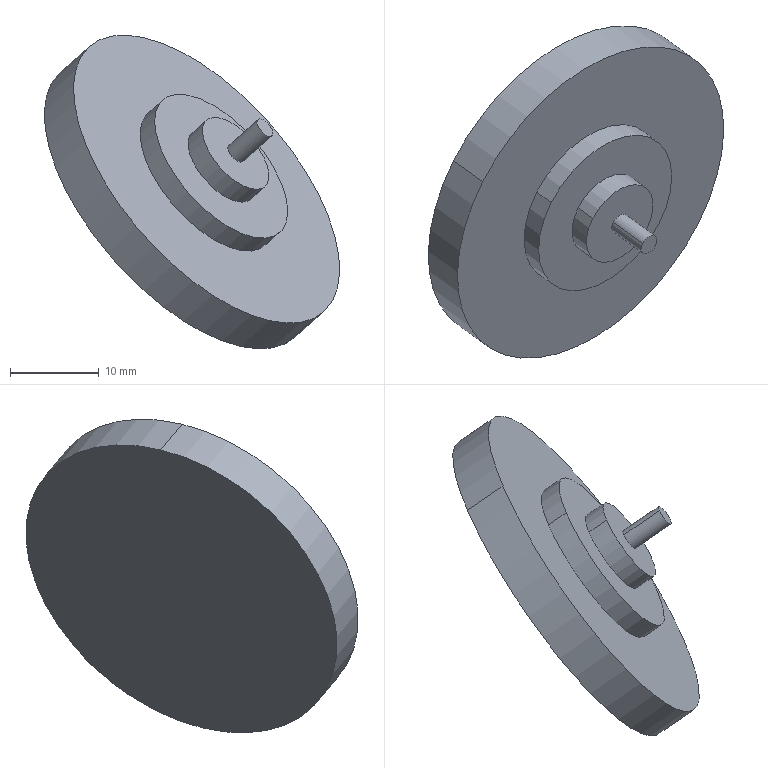Component | SolidWorks | ConnectingPlate-1 | 1 solid | 13 faces | box 33.37 x 37.55 x 35.44 mm | volume 7288 mm3 | cylinder 8 | plane 5 | commonest cylinder face diameters 2.4 x2 10 x2 20 x2 40 x2 | material Copper
build123d program:
from build123d import *

# Parameters (mm, degrees)
SKETCH2_R           = 20
BOSS_EXTRUDE1_DEPTH = 5
SKETCH2_4_R         = 10
BOSS_EXTRUDE2_DEPTH = 2.5
SKETCH2_5_R         = 5
BOSS_EXTRUDE3_DEPTH = 5
SKETCH2_6_R         = 1.2
BOSS_EXTRUDE4_DEPTH = 10


with BuildPart() as part:
    # Sketch2 → Boss-Extrude1 (new body)
    with BuildSketch(Plane(origin=(0, 0, 0), x_dir=(1, 0, 0), z_dir=(0, 1, 0))):
        with Locations(Location((0, 0, 0), (0, 0, 270))):
            Circle(SKETCH2_R)
    extrude(amount=BOSS_EXTRUDE1_DEPTH)

    # Sketch2_4 → Boss-Extrude2 (add)
    with BuildSketch(Plane(origin=(0, 0, 0), x_dir=(1, 0, 0), z_dir=(0, 1, 0))):
        with Locations(Location((0, 0, 0), (0, 0, 270))):
            Circle(SKETCH2_4_R)
    extrude(amount=-BOSS_EXTRUDE2_DEPTH)

    # Sketch2_5 → Boss-Extrude3 (add)
    with BuildSketch(Plane(origin=(0, 0, 0), x_dir=(1, 0, 0), z_dir=(0, 1, 0))):
        with Locations(Location((0, 0, 0), (0, 0, 270))):
            Circle(SKETCH2_5_R)
    extrude(amount=-BOSS_EXTRUDE3_DEPTH)

    # Sketch2_6 → Boss-Extrude4 (add)
    with BuildSketch(Plane(origin=(0, 0, 0), x_dir=(1, 0, 0), z_dir=(0, 1, 0))):
        with Locations(Location((0, 0, 0), (0, 0, 270))):
            Circle(SKETCH2_6_R)
    extrude(amount=-BOSS_EXTRUDE4_DEPTH)


solid = part.part

# Placed as in the assembly
solid = solid.moved(Location((-327.305, -1538.595, -15.587), (-73.169, 23.56, 45.986)))
STEP:
#1=COLOUR_RGB('',0.7922,0.8196,0.9333);
#2=FILL_AREA_STYLE_COLOUR('',#1);
#3=FILL_AREA_STYLE('',(#2));
#4=SURFACE_STYLE_FILL_AREA(#3);
#5=SURFACE_SIDE_STYLE('',(#4));
#6=SURFACE_STYLE_USAGE(.BOTH.,#5);
#7=PRESENTATION_STYLE_ASSIGNMENT((#6));
#8=CARTESIAN_POINT('',(-12.598,-60.768,-0.4217));
#9=VERTEX_POINT('',#8);
#10=CARTESIAN_POINT('',(-12.655,-60.757,-0.3475));
#11=VERTEX_POINT('',#10);
#12=CARTESIAN_POINT('',(-12.626,-60.762,-0.3846));
#13=DIRECTION('',(-0.6592,0.4763,-0.5818));
#14=DIRECTION('',(0.6087,-0.1163,-0.7848));
#15=AXIS2_PLACEMENT_3D('',#12,#13,#14);
#16=CIRCLE('',#15,0.04724);
#17=EDGE_CURVE('',#9,#11,#16,.T.);
#18=ORIENTED_EDGE('',*,*,#17,.T.);
#19=CARTESIAN_POINT('',(-12.785,-60.663,-0.4621));
#20=VERTEX_POINT('',#19);
#21=CARTESIAN_POINT('',(-12.655,-60.757,-0.3475));
#22=DIRECTION('',(-0.6592,0.4763,-0.5818));
#23=VECTOR('',#22,39.37);
#24=LINE('',#21,#23);
#25=EDGE_CURVE('',#11,#20,#24,.T.);
#26=ORIENTED_EDGE('',*,*,#25,.T.);
#27=CARTESIAN_POINT('',(-12.727,-60.674,-0.5362));
#28=VERTEX_POINT('',#27);
#29=CARTESIAN_POINT('',(-12.756,-60.668,-0.4991));
#30=DIRECTION('',(-0.6592,0.4763,-0.5818));
#31=DIRECTION('',(0.6087,-0.1163,-0.7848));
#32=AXIS2_PLACEMENT_3D('',#29,#30,#31);
#33=CIRCLE('',#32,0.04724);
#34=EDGE_CURVE('',#28,#20,#33,.T.);
#35=ORIENTED_EDGE('',*,*,#34,.F.);
#36=CARTESIAN_POINT('',(-12.598,-60.768,-0.4217));
#37=DIRECTION('',(-0.6592,0.4763,-0.5818));
#38=VECTOR('',#37,39.37);
#39=LINE('',#36,#38);
#40=EDGE_CURVE('',#9,#28,#39,.T.);
#41=ORIENTED_EDGE('',*,*,#40,.F.);
#42=EDGE_LOOP('',(#18,#26,#35,#41));
#43=FACE_OUTER_BOUND('',#42,.T.);
#44=CARTESIAN_POINT('',(-12.626,-60.762,-0.3846));
#45=DIRECTION('',(-0.6592,0.4763,-0.5818));
#46=DIRECTION('',(0.6087,-0.1163,-0.7848));
#47=AXIS2_PLACEMENT_3D('',#44,#45,#46);
#48=CYLINDRICAL_SURFACE('',#47,0.04724);
#49=ADVANCED_FACE('',(#43),#48,.T.);
#50=CARTESIAN_POINT('',(-12.636,-60.691,-0.6536));
#51=VERTEX_POINT('',#50);
#52=CARTESIAN_POINT('',(-12.876,-60.645,-0.3446));
#53=VERTEX_POINT('',#52);
#54=CARTESIAN_POINT('',(-12.756,-60.668,-0.4991));
#55=DIRECTION('',(-0.6592,0.4763,-0.5818));
#56=DIRECTION('',(0.6087,-0.1163,-0.7848));
#57=AXIS2_PLACEMENT_3D('',#54,#55,#56);
#58=CIRCLE('',#57,0.1969);
#59=EDGE_CURVE('',#51,#53,#58,.T.);
#60=ORIENTED_EDGE('',*,*,#59,.T.);
#61=CARTESIAN_POINT('',(-12.941,-60.599,-0.4019));
#62=VERTEX_POINT('',#61);
#63=CARTESIAN_POINT('',(-12.876,-60.645,-0.3446));
#64=DIRECTION('',(-0.6592,0.4763,-0.5818));
#65=VECTOR('',#64,39.37);
#66=LINE('',#63,#65);
#67=EDGE_CURVE('',#53,#62,#66,.T.);
#68=ORIENTED_EDGE('',*,*,#67,.T.);
#69=CARTESIAN_POINT('',(-12.701,-60.644,-0.7109));
#70=VERTEX_POINT('',#69);
#71=CARTESIAN_POINT('',(-12.821,-60.622,-0.5564));
#72=DIRECTION('',(-0.6592,0.4763,-0.5818));
#73=DIRECTION('',(0.6087,-0.1163,-0.7848));
#74=AXIS2_PLACEMENT_3D('',#71,#72,#73);
#75=CIRCLE('',#74,0.1969);
#76=EDGE_CURVE('',#70,#62,#75,.T.);
#77=ORIENTED_EDGE('',*,*,#76,.F.);
#78=CARTESIAN_POINT('',(-12.636,-60.691,-0.6536));
#79=DIRECTION('',(-0.6592,0.4763,-0.5818));
#80=VECTOR('',#79,39.37);
#81=LINE('',#78,#80);
#82=EDGE_CURVE('',#51,#70,#81,.T.);
#83=ORIENTED_EDGE('',*,*,#82,.F.);
#84=EDGE_LOOP('',(#60,#68,#77,#83));
#85=FACE_OUTER_BOUND('',#84,.T.);
#86=CARTESIAN_POINT('',(-12.756,-60.668,-0.4991));
#87=DIRECTION('',(-0.6592,0.4763,-0.5818));
#88=DIRECTION('',(0.6087,-0.1163,-0.7848));
#89=AXIS2_PLACEMENT_3D('',#86,#87,#88);
#90=CYLINDRICAL_SURFACE('',#89,0.1969);
#91=ADVANCED_FACE('',(#85),#90,.T.);
#92=CARTESIAN_POINT('',(-12.581,-60.667,-0.8654));
#93=VERTEX_POINT('',#92);
#94=CARTESIAN_POINT('',(-13.061,-60.576,-0.2474));
#95=VERTEX_POINT('',#94);
#96=CARTESIAN_POINT('',(-12.821,-60.622,-0.5564));
#97=DIRECTION('',(-0.6592,0.4763,-0.5818));
#98=DIRECTION('',(0.6087,-0.1163,-0.7848));
#99=AXIS2_PLACEMENT_3D('',#96,#97,#98);
#100=CIRCLE('',#99,0.3937);
#101=EDGE_CURVE('',#93,#95,#100,.T.);
#102=ORIENTED_EDGE('',*,*,#101,.T.);
#103=CARTESIAN_POINT('',(-13.126,-60.529,-0.3047));
#104=VERTEX_POINT('',#103);
#105=CARTESIAN_POINT('',(-13.061,-60.576,-0.2474));
#106=DIRECTION('',(-0.6592,0.4763,-0.5818));
#107=VECTOR('',#106,39.37);
#108=LINE('',#105,#107);
#109=EDGE_CURVE('',#95,#104,#108,.T.);
#110=ORIENTED_EDGE('',*,*,#109,.T.);
#111=CARTESIAN_POINT('',(-12.646,-60.62,-0.9227));
#112=VERTEX_POINT('',#111);
#113=CARTESIAN_POINT('',(-12.886,-60.575,-0.6137));
#114=DIRECTION('',(-0.6592,0.4763,-0.5818));
#115=DIRECTION('',(0.6087,-0.1163,-0.7848));
#116=AXIS2_PLACEMENT_3D('',#113,#114,#115);
#117=CIRCLE('',#116,0.3937);
#118=EDGE_CURVE('',#112,#104,#117,.T.);
#119=ORIENTED_EDGE('',*,*,#118,.F.);
#120=CARTESIAN_POINT('',(-12.581,-60.667,-0.8654));
#121=DIRECTION('',(-0.6592,0.4763,-0.5818));
#122=VECTOR('',#121,39.37);
#123=LINE('',#120,#122);
#124=EDGE_CURVE('',#93,#112,#123,.T.);
#125=ORIENTED_EDGE('',*,*,#124,.F.);
#126=EDGE_LOOP('',(#102,#110,#119,#125));
#127=FACE_OUTER_BOUND('',#126,.T.);
#128=CARTESIAN_POINT('',(-12.821,-60.622,-0.5564));
#129=DIRECTION('',(-0.6592,0.4763,-0.5818));
#130=DIRECTION('',(0.6087,-0.1163,-0.7848));
#131=AXIS2_PLACEMENT_3D('',#128,#129,#130);
#132=CYLINDRICAL_SURFACE('',#131,0.3937);
#133=ADVANCED_FACE('',(#127),#132,.T.);
#134=CARTESIAN_POINT('',(-12.536,-60.572,-1.346));
#135=VERTEX_POINT('',#134);
#136=CARTESIAN_POINT('',(-13.495,-60.389,-0.1102));
#137=VERTEX_POINT('',#136);
#138=CARTESIAN_POINT('',(-13.016,-60.481,-0.7282));
#139=DIRECTION('',(-0.6592,0.4763,-0.5818));
#140=DIRECTION('',(0.6087,-0.1163,-0.7848));
#141=AXIS2_PLACEMENT_3D('',#138,#139,#140);
#142=CIRCLE('',#141,0.7874);
#143=EDGE_CURVE('',#135,#137,#142,.T.);
#144=ORIENTED_EDGE('',*,*,#143,.F.);
#145=CARTESIAN_POINT('',(-12.407,-60.666,-1.232));
#146=VERTEX_POINT('',#145);
#147=CARTESIAN_POINT('',(-12.536,-60.572,-1.346));
#148=DIRECTION('',(0.6592,-0.4763,0.5818));
#149=VECTOR('',#148,39.37);
#150=LINE('',#147,#149);
#151=EDGE_CURVE('',#135,#146,#150,.T.);
#152=ORIENTED_EDGE('',*,*,#151,.T.);
#153=CARTESIAN_POINT('',(-13.365,-60.483,0.00431));
#154=VERTEX_POINT('',#153);
#155=CARTESIAN_POINT('',(-12.886,-60.575,-0.6137));
#156=DIRECTION('',(-0.6592,0.4763,-0.5818));
#157=DIRECTION('',(0.6087,-0.1163,-0.7848));
#158=AXIS2_PLACEMENT_3D('',#155,#156,#157);
#159=CIRCLE('',#158,0.7874);
#160=EDGE_CURVE('',#146,#154,#159,.T.);
#161=ORIENTED_EDGE('',*,*,#160,.T.);
#162=CARTESIAN_POINT('',(-13.495,-60.389,-0.1102));
#163=DIRECTION('',(0.6592,-0.4763,0.5818));
#164=VECTOR('',#163,39.37);
#165=LINE('',#162,#164);
#166=EDGE_CURVE('',#137,#154,#165,.T.);
#167=ORIENTED_EDGE('',*,*,#166,.F.);
#168=EDGE_LOOP('',(#144,#152,#161,#167));
#169=FACE_OUTER_BOUND('',#168,.T.);
#170=CARTESIAN_POINT('',(-13.016,-60.481,-0.7282));
#171=DIRECTION('',(0.6592,-0.4763,0.5818));
#172=DIRECTION('',(-0.6087,0.1163,0.7848));
#173=AXIS2_PLACEMENT_3D('',#170,#171,#172);
#174=CYLINDRICAL_SURFACE('',#173,0.7874);
#175=ADVANCED_FACE('',(#169),#174,.T.);
#176=ORIENTED_EDGE('',*,*,#151,.F.);
#177=CARTESIAN_POINT('',(-13.016,-60.481,-0.7282));
#178=DIRECTION('',(-0.6592,0.4763,-0.5818));
#179=DIRECTION('',(0.6087,-0.1163,-0.7848));
#180=AXIS2_PLACEMENT_3D('',#177,#178,#179);
#181=CIRCLE('',#180,0.7874);
#182=EDGE_CURVE('',#137,#135,#181,.T.);
#183=ORIENTED_EDGE('',*,*,#182,.F.);
#184=ORIENTED_EDGE('',*,*,#166,.T.);
#185=CARTESIAN_POINT('',(-12.886,-60.575,-0.6137));
#186=DIRECTION('',(-0.6592,0.4763,-0.5818));
#187=DIRECTION('',(0.6087,-0.1163,-0.7848));
#188=AXIS2_PLACEMENT_3D('',#185,#186,#187);
#189=CIRCLE('',#188,0.7874);
#190=EDGE_CURVE('',#154,#146,#189,.T.);
#191=ORIENTED_EDGE('',*,*,#190,.T.);
#192=EDGE_LOOP('',(#176,#183,#184,#191));
#193=FACE_OUTER_BOUND('',#192,.T.);
#194=CARTESIAN_POINT('',(-13.016,-60.481,-0.7282));
#195=DIRECTION('',(0.6592,-0.4763,0.5818));
#196=DIRECTION('',(-0.6087,0.1163,0.7848));
#197=AXIS2_PLACEMENT_3D('',#194,#195,#196);
#198=CYLINDRICAL_SURFACE('',#197,0.7874);
#199=ADVANCED_FACE('',(#193),#198,.T.);
#200=ORIENTED_EDGE('',*,*,#182,.T.);
#201=ORIENTED_EDGE('',*,*,#143,.T.);
#202=EDGE_LOOP('',(#200,#201));
#203=FACE_OUTER_BOUND('',#202,.T.);
#204=CARTESIAN_POINT('',(-13.016,-60.481,-0.7282));
#205=DIRECTION('',(-0.6592,0.4763,-0.5818));
#206=DIRECTION('',(0.6087,-0.1163,-0.7848));
#207=AXIS2_PLACEMENT_3D('',#204,#205,#206);
#208=PLANE('',#207);
#209=ADVANCED_FACE('',(#203),#208,.T.);
#210=ORIENTED_EDGE('',*,*,#118,.T.);
#211=CARTESIAN_POINT('',(-12.886,-60.575,-0.6137));
#212=DIRECTION('',(-0.6592,0.4763,-0.5818));
#213=DIRECTION('',(0.6087,-0.1163,-0.7848));
#214=AXIS2_PLACEMENT_3D('',#211,#212,#213);
#215=CIRCLE('',#214,0.3937);
#216=EDGE_CURVE('',#104,#112,#215,.T.);
#217=ORIENTED_EDGE('',*,*,#216,.T.);
#218=EDGE_LOOP('',(#210,#217));
#219=FACE_BOUND('',#218,.T.);
#220=ORIENTED_EDGE('',*,*,#190,.F.);
#221=ORIENTED_EDGE('',*,*,#160,.F.);
#222=EDGE_LOOP('',(#220,#221));
#223=FACE_OUTER_BOUND('',#222,.T.);
#224=CARTESIAN_POINT('',(-12.886,-60.575,-0.6137));
#225=DIRECTION('',(-0.6592,0.4763,-0.5818));
#226=DIRECTION('',(0.6087,-0.1163,-0.7848));
#227=AXIS2_PLACEMENT_3D('',#224,#225,#226);
#228=PLANE('',#227);
#229=ADVANCED_FACE('',(#219,#223),#228,.F.);
#230=ORIENTED_EDGE('',*,*,#109,.F.);
#231=CARTESIAN_POINT('',(-12.821,-60.622,-0.5564));
#232=DIRECTION('',(-0.6592,0.4763,-0.5818));
#233=DIRECTION('',(0.6087,-0.1163,-0.7848));
#234=AXIS2_PLACEMENT_3D('',#231,#232,#233);
#235=CIRCLE('',#234,0.3937);
#236=EDGE_CURVE('',#95,#93,#235,.T.);
#237=ORIENTED_EDGE('',*,*,#236,.T.);
#238=ORIENTED_EDGE('',*,*,#124,.T.);
#239=ORIENTED_EDGE('',*,*,#216,.F.);
#240=EDGE_LOOP('',(#230,#237,#238,#239));
#241=FACE_OUTER_BOUND('',#240,.T.);
#242=CARTESIAN_POINT('',(-12.821,-60.622,-0.5564));
#243=DIRECTION('',(-0.6592,0.4763,-0.5818));
#244=DIRECTION('',(0.6087,-0.1163,-0.7848));
#245=AXIS2_PLACEMENT_3D('',#242,#243,#244);
#246=CYLINDRICAL_SURFACE('',#245,0.3937);
#247=ADVANCED_FACE('',(#241),#246,.T.);
#248=ORIENTED_EDGE('',*,*,#76,.T.);
#249=CARTESIAN_POINT('',(-12.821,-60.622,-0.5564));
#250=DIRECTION('',(-0.6592,0.4763,-0.5818));
#251=DIRECTION('',(0.6087,-0.1163,-0.7848));
#252=AXIS2_PLACEMENT_3D('',#249,#250,#251);
#253=CIRCLE('',#252,0.1969);
#254=EDGE_CURVE('',#62,#70,#253,.T.);
#255=ORIENTED_EDGE('',*,*,#254,.T.);
#256=EDGE_LOOP('',(#248,#255));
#257=FACE_BOUND('',#256,.T.);
#258=ORIENTED_EDGE('',*,*,#101,.F.);
#259=ORIENTED_EDGE('',*,*,#236,.F.);
#260=EDGE_LOOP('',(#258,#259));
#261=FACE_OUTER_BOUND('',#260,.T.);
#262=CARTESIAN_POINT('',(-12.821,-60.622,-0.5564));
#263=DIRECTION('',(-0.6592,0.4763,-0.5818));
#264=DIRECTION('',(0.6087,-0.1163,-0.7848));
#265=AXIS2_PLACEMENT_3D('',#262,#263,#264);
#266=PLANE('',#265);
#267=ADVANCED_FACE('',(#257,#261),#266,.F.);
#268=ORIENTED_EDGE('',*,*,#67,.F.);
#269=CARTESIAN_POINT('',(-12.756,-60.668,-0.4991));
#270=DIRECTION('',(-0.6592,0.4763,-0.5818));
#271=DIRECTION('',(0.6087,-0.1163,-0.7848));
#272=AXIS2_PLACEMENT_3D('',#269,#270,#271);
#273=CIRCLE('',#272,0.1969);
#274=EDGE_CURVE('',#53,#51,#273,.T.);
#275=ORIENTED_EDGE('',*,*,#274,.T.);
#276=ORIENTED_EDGE('',*,*,#82,.T.);
#277=ORIENTED_EDGE('',*,*,#254,.F.);
#278=EDGE_LOOP('',(#268,#275,#276,#277));
#279=FACE_OUTER_BOUND('',#278,.T.);
#280=CARTESIAN_POINT('',(-12.756,-60.668,-0.4991));
#281=DIRECTION('',(-0.6592,0.4763,-0.5818));
#282=DIRECTION('',(0.6087,-0.1163,-0.7848));
#283=AXIS2_PLACEMENT_3D('',#280,#281,#282);
#284=CYLINDRICAL_SURFACE('',#283,0.1969);
#285=ADVANCED_FACE('',(#279),#284,.T.);
#286=ORIENTED_EDGE('',*,*,#34,.T.);
#287=CARTESIAN_POINT('',(-12.756,-60.668,-0.4991));
#288=DIRECTION('',(-0.6592,0.4763,-0.5818));
#289=DIRECTION('',(0.6087,-0.1163,-0.7848));
#290=AXIS2_PLACEMENT_3D('',#287,#288,#289);
#291=CIRCLE('',#290,0.04724);
#292=EDGE_CURVE('',#20,#28,#291,.T.);
#293=ORIENTED_EDGE('',*,*,#292,.T.);
#294=EDGE_LOOP('',(#286,#293));
#295=FACE_BOUND('',#294,.T.);
#296=ORIENTED_EDGE('',*,*,#59,.F.);
#297=ORIENTED_EDGE('',*,*,#274,.F.);
#298=EDGE_LOOP('',(#296,#297));
#299=FACE_OUTER_BOUND('',#298,.T.);
#300=CARTESIAN_POINT('',(-12.756,-60.668,-0.4991));
#301=DIRECTION('',(-0.6592,0.4763,-0.5818));
#302=DIRECTION('',(0.6087,-0.1163,-0.7848));
#303=AXIS2_PLACEMENT_3D('',#300,#301,#302);
#304=PLANE('',#303);
#305=ADVANCED_FACE('',(#295,#299),#304,.F.);
#306=ORIENTED_EDGE('',*,*,#25,.F.);
#307=CARTESIAN_POINT('',(-12.626,-60.762,-0.3846));
#308=DIRECTION('',(-0.6592,0.4763,-0.5818));
#309=DIRECTION('',(0.6087,-0.1163,-0.7848));
#310=AXIS2_PLACEMENT_3D('',#307,#308,#309);
#311=CIRCLE('',#310,0.04724);
#312=EDGE_CURVE('',#11,#9,#311,.T.);
#313=ORIENTED_EDGE('',*,*,#312,.T.);
#314=ORIENTED_EDGE('',*,*,#40,.T.);
#315=ORIENTED_EDGE('',*,*,#292,.F.);
#316=EDGE_LOOP('',(#306,#313,#314,#315));
#317=FACE_OUTER_BOUND('',#316,.T.);
#318=CARTESIAN_POINT('',(-12.626,-60.762,-0.3846));
#319=DIRECTION('',(-0.6592,0.4763,-0.5818));
#320=DIRECTION('',(0.6087,-0.1163,-0.7848));
#321=AXIS2_PLACEMENT_3D('',#318,#319,#320);
#322=CYLINDRICAL_SURFACE('',#321,0.04724);
#323=ADVANCED_FACE('',(#317),#322,.T.);
#324=ORIENTED_EDGE('',*,*,#17,.F.);
#325=ORIENTED_EDGE('',*,*,#312,.F.);
#326=EDGE_LOOP('',(#324,#325));
#327=FACE_OUTER_BOUND('',#326,.T.);
#328=CARTESIAN_POINT('',(-12.626,-60.762,-0.3846));
#329=DIRECTION('',(-0.6592,0.4763,-0.5818));
#330=DIRECTION('',(0.6087,-0.1163,-0.7848));
#331=AXIS2_PLACEMENT_3D('',#328,#329,#330);
#332=PLANE('',#331);
#333=ADVANCED_FACE('',(#327),#332,.F.);
#334=CLOSED_SHELL('',(#49,#91,#133,#175,#199,#209,#229,#247,#267,#285,#305,#323,#333));
#335=MANIFOLD_SOLID_BREP('',#334);
#336=STYLED_ITEM('',(#7),#335);
#337=(LENGTH_UNIT()NAMED_UNIT(*)SI_UNIT($,.METRE.));
#338=LENGTH_MEASURE_WITH_UNIT(LENGTH_MEASURE(0.0254),#337);
#339=DIMENSIONAL_EXPONENTS(1.,0.,0.,0.,0.,0.,0.);
#340=(CONVERSION_BASED_UNIT('',#338)LENGTH_UNIT()NAMED_UNIT(#339));
#341=UNCERTAINTY_MEASURE_WITH_UNIT(LENGTH_MEASURE(0.00001),#340,'','');
#342=(NAMED_UNIT(*)PLANE_ANGLE_UNIT()SI_UNIT($,.RADIAN.));
#343=(NAMED_UNIT(*)SI_UNIT($,.STERADIAN.)SOLID_ANGLE_UNIT());
#344=(GEOMETRIC_REPRESENTATION_CONTEXT(3)GLOBAL_UNCERTAINTY_ASSIGNED_CONTEXT((#341))GLOBAL_UNIT_ASSIGNED_CONTEXT((#340,#342,#343))REPRESENTATION_CONTEXT('',''));
#345=MECHANICAL_DESIGN_GEOMETRIC_PRESENTATION_REPRESENTATION('',(#336),#344);
#346=CARTESIAN_POINT('',(0.,0.,0.));
#347=DIRECTION('',(0.,0.,1.));
#348=DIRECTION('',(1.,0.,0.));
#349=AXIS2_PLACEMENT_3D('',#346,#347,#348);
#350=(LENGTH_UNIT()NAMED_UNIT(*)SI_UNIT($,.METRE.));
#351=LENGTH_MEASURE_WITH_UNIT(LENGTH_MEASURE(0.0254),#350);
#352=DIMENSIONAL_EXPONENTS(1.,0.,0.,0.,0.,0.,0.);
#353=(CONVERSION_BASED_UNIT('',#351)LENGTH_UNIT()NAMED_UNIT(#352));
#354=UNCERTAINTY_MEASURE_WITH_UNIT(LENGTH_MEASURE(0.00001),#353,'','');
#355=(NAMED_UNIT(*)PLANE_ANGLE_UNIT()SI_UNIT($,.RADIAN.));
#356=(NAMED_UNIT(*)SI_UNIT($,.STERADIAN.)SOLID_ANGLE_UNIT());
#357=(GEOMETRIC_REPRESENTATION_CONTEXT(3)GLOBAL_UNCERTAINTY_ASSIGNED_CONTEXT((#354))GLOBAL_UNIT_ASSIGNED_CONTEXT((#353,#355,#356))REPRESENTATION_CONTEXT('',''));
#358=ADVANCED_BREP_SHAPE_REPRESENTATION('',(#335,#349),#357);
#359=PRESENTATION_LAYER_ASSIGNMENT('','',(#336));